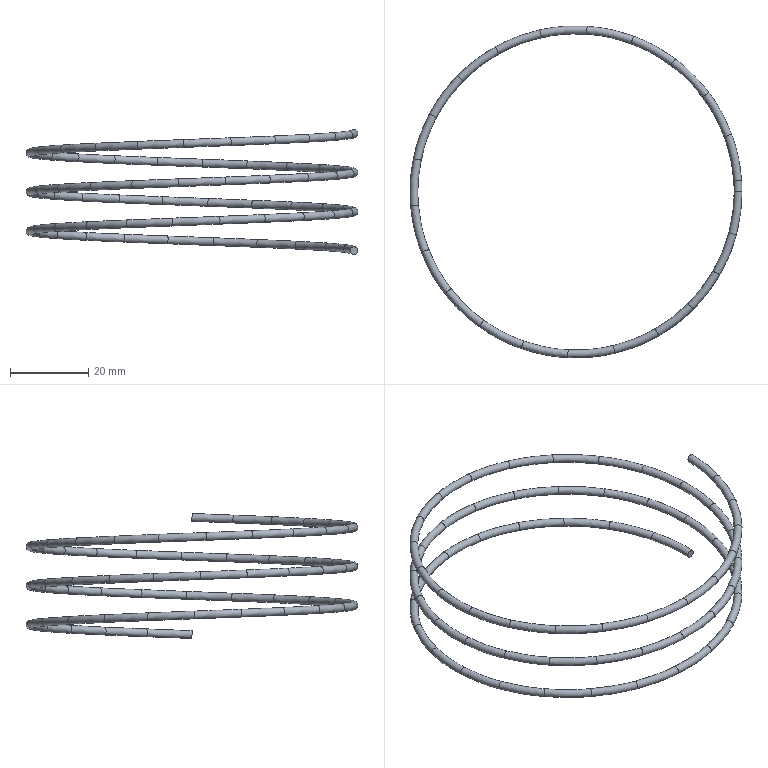Component | NX | CH3404_10-5 | 1 solid | 68 faces | volume 2459 mm3 | torus 66 | plane 2